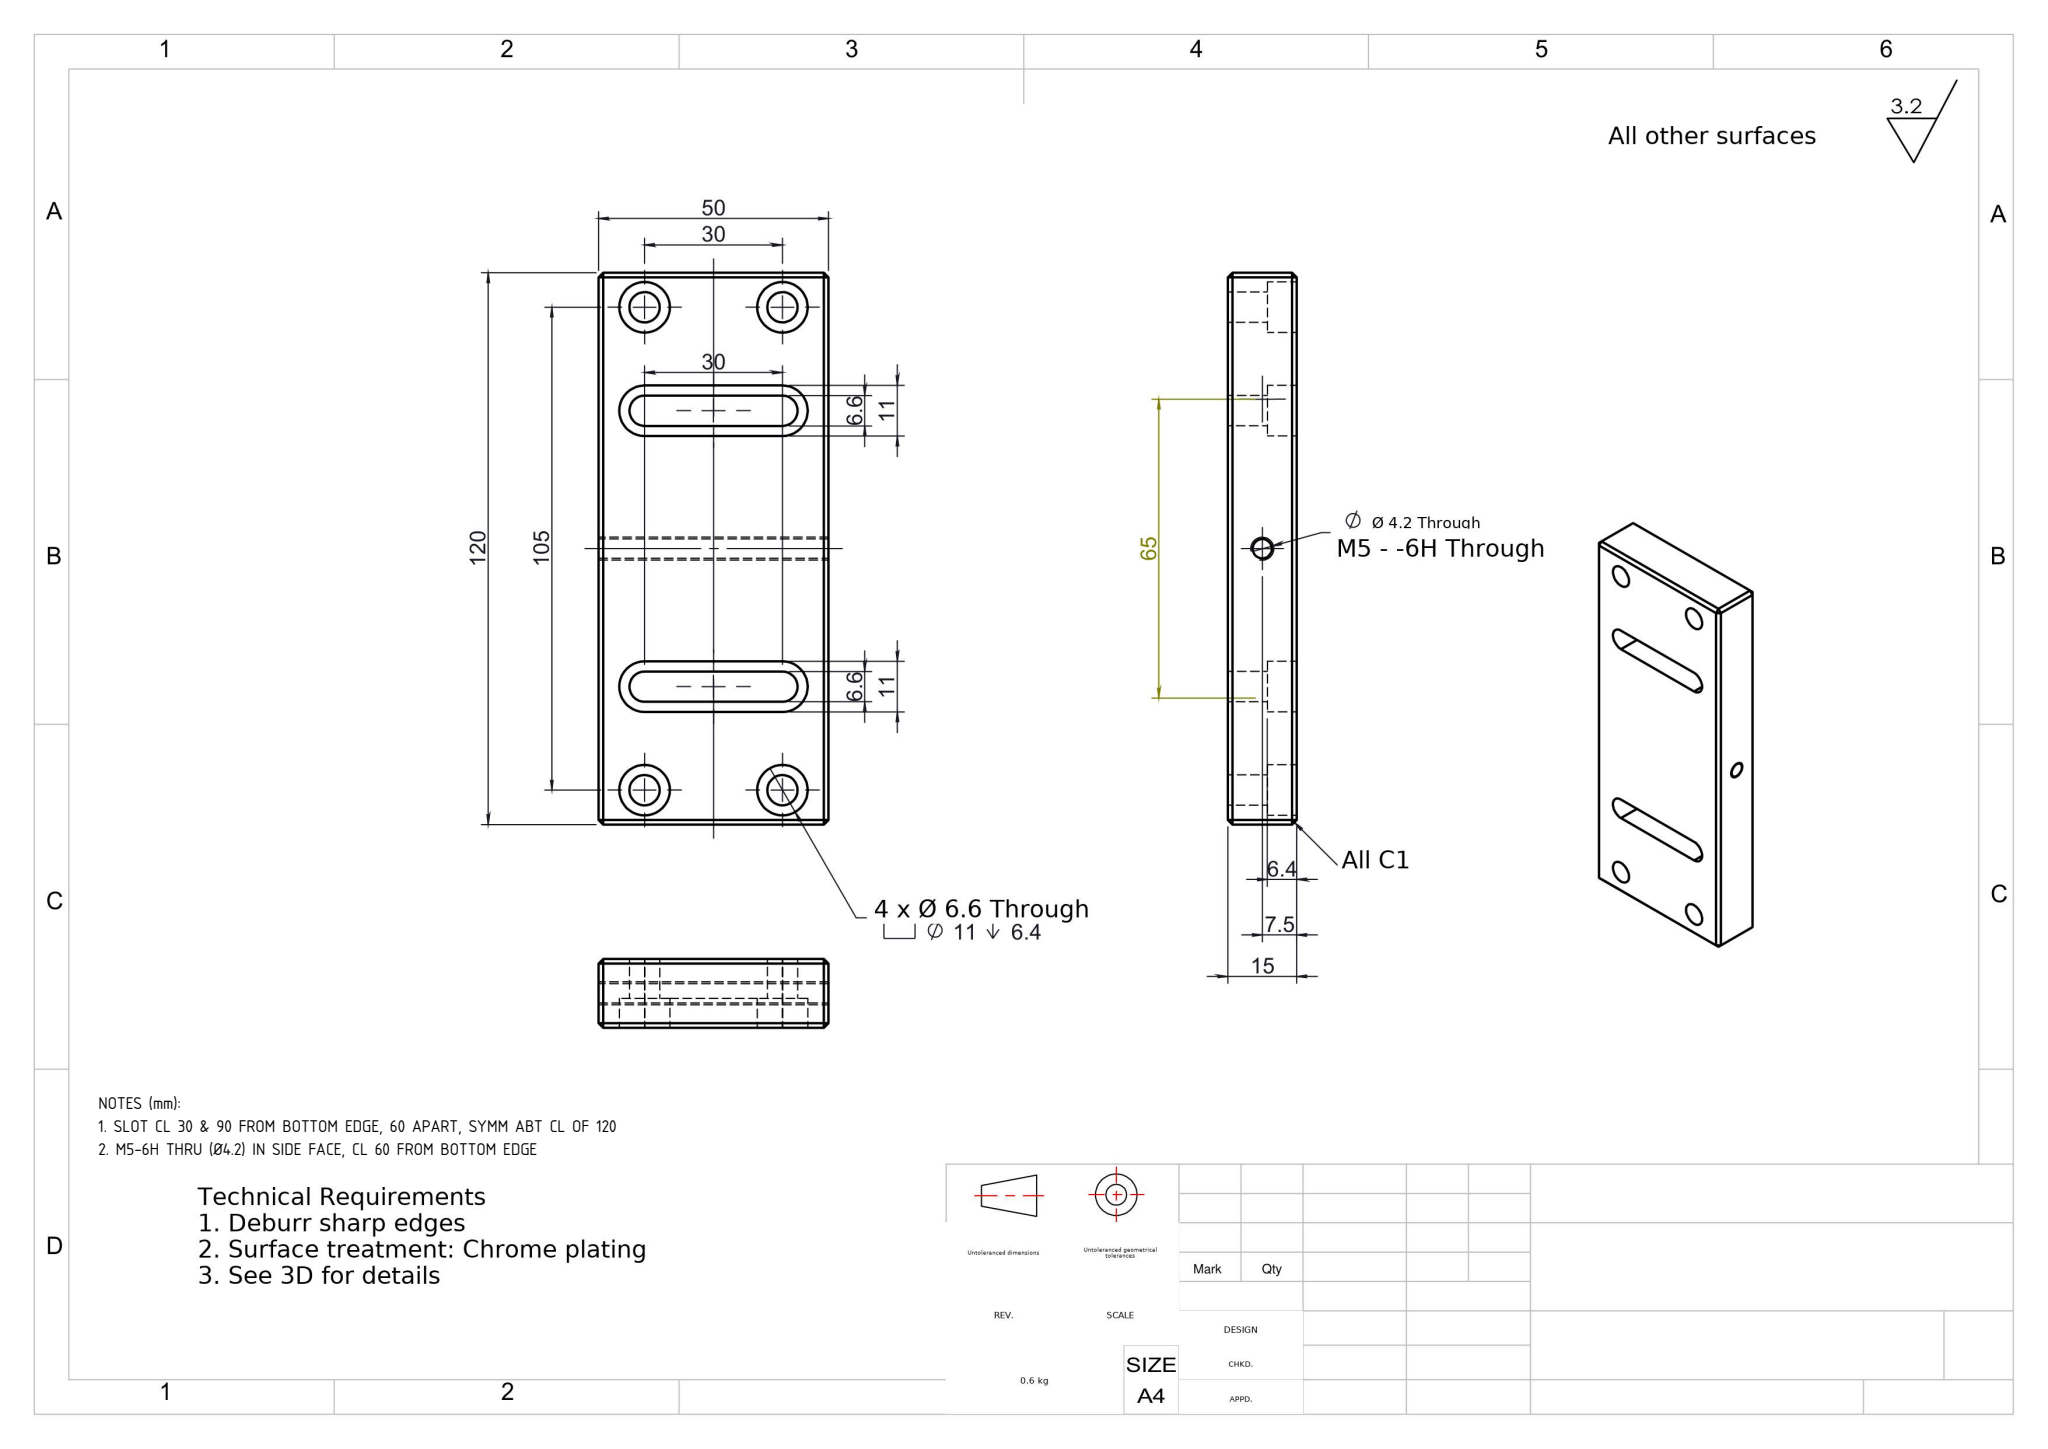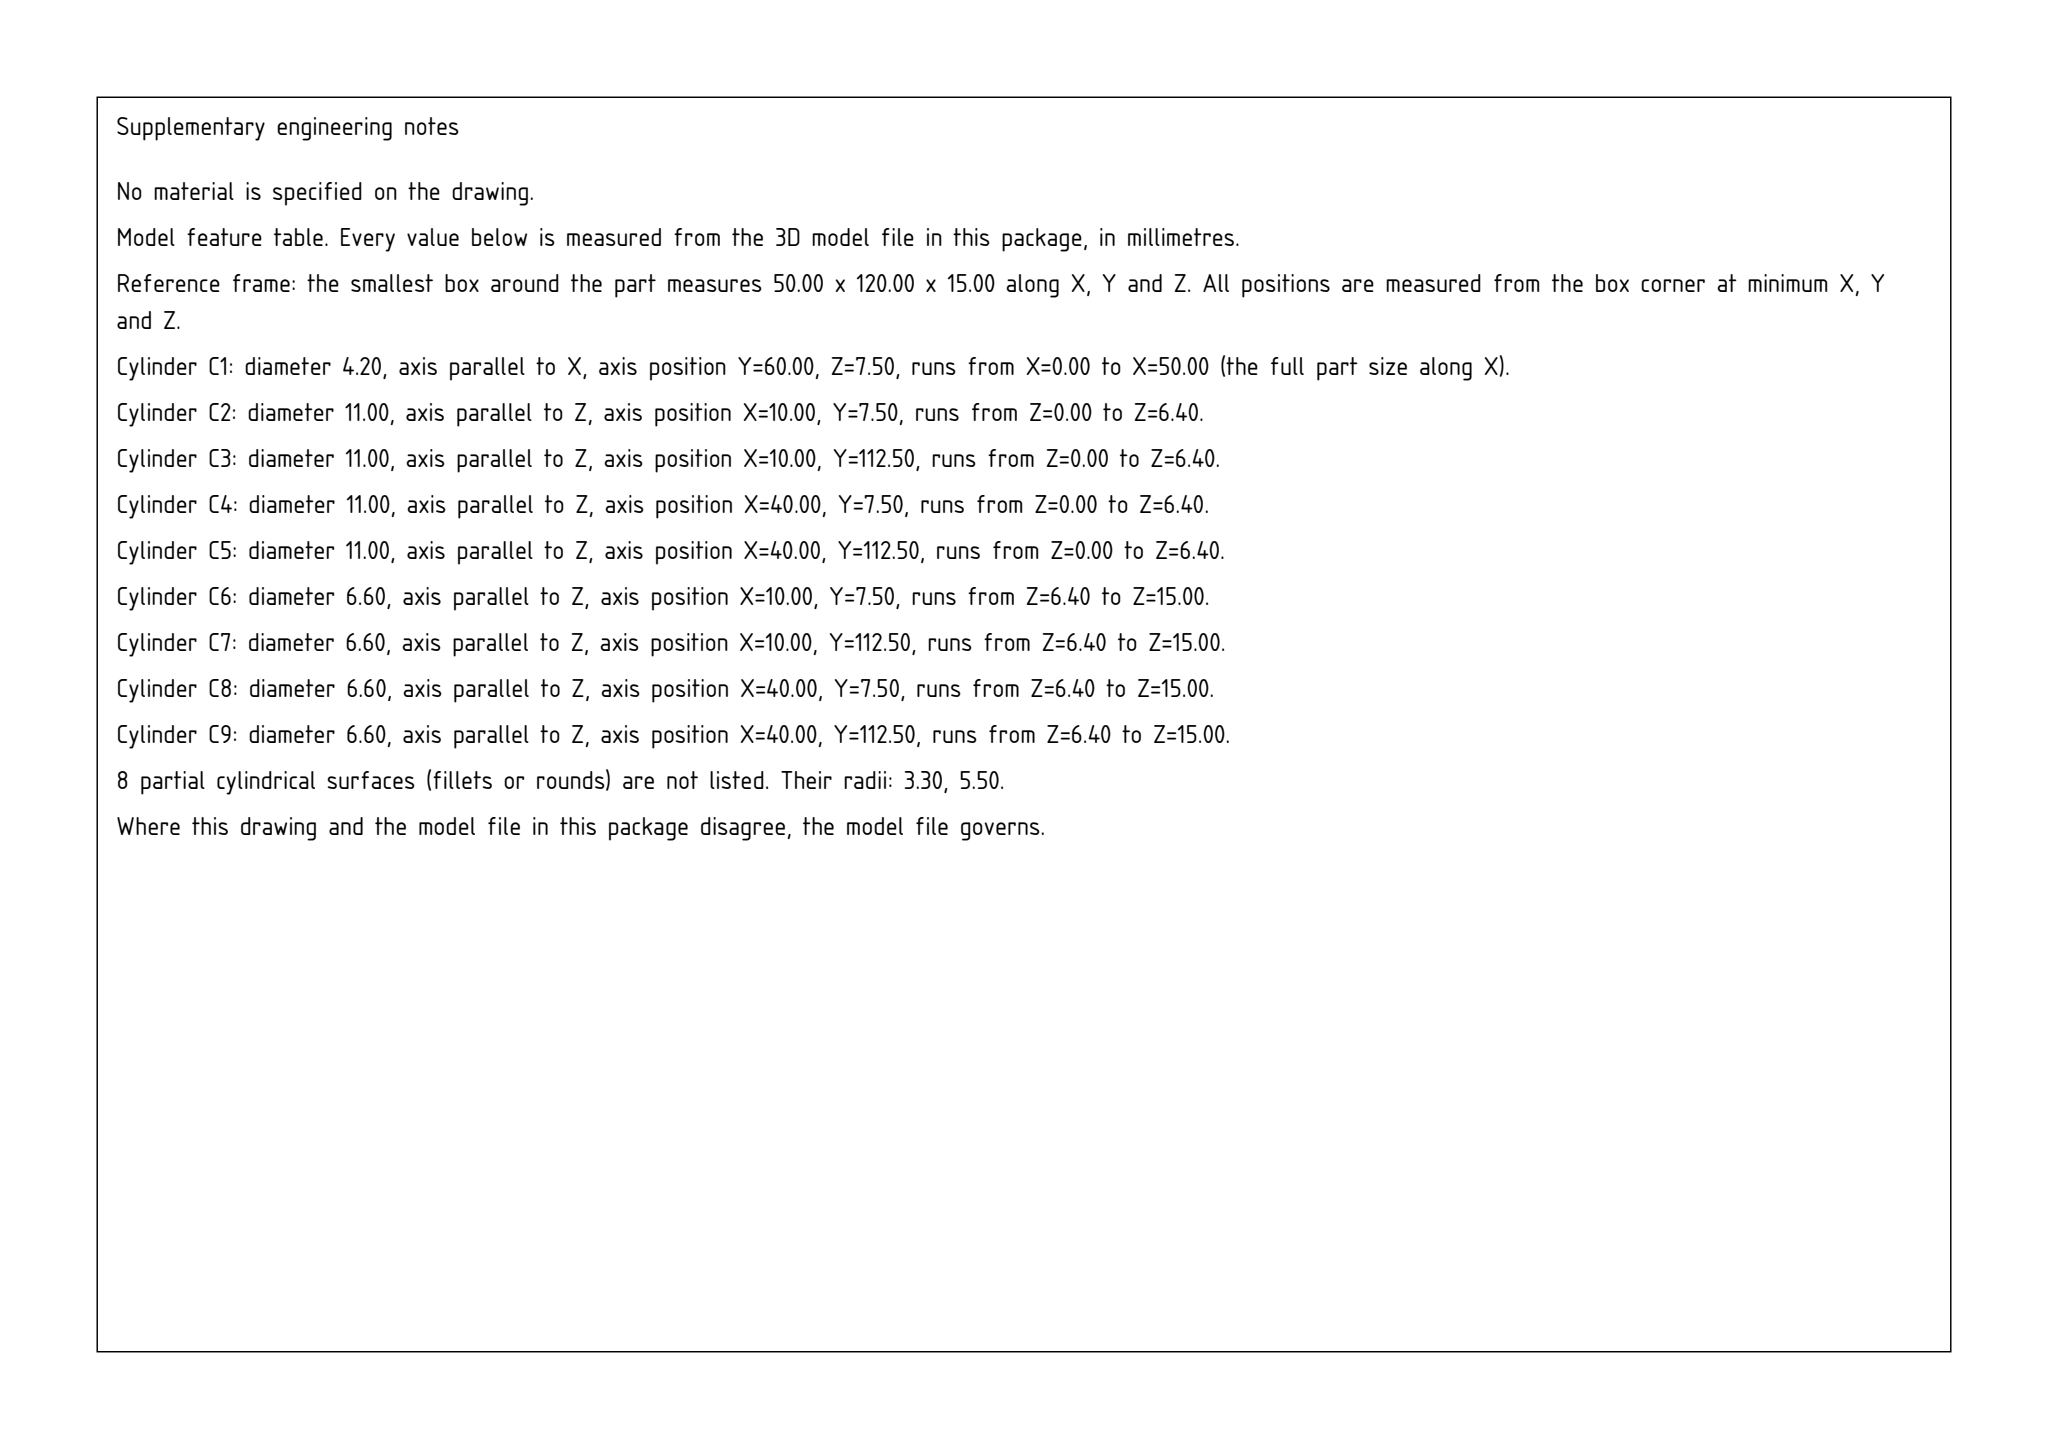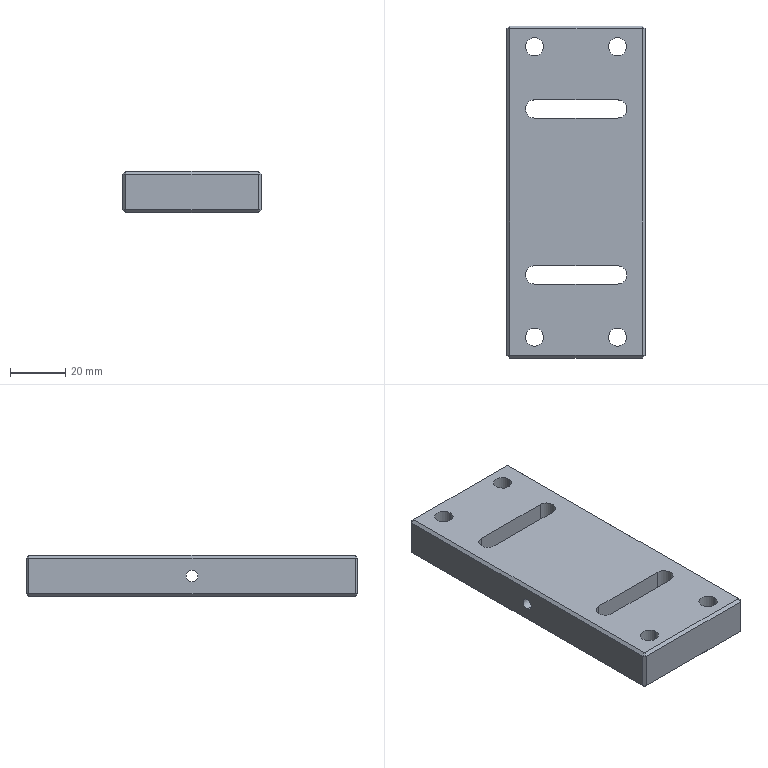Part | SolidWorks | mm | 1 solid | 70 faces | box 50 x 120 x 15 mm | volume 75898 mm3 | plane 40 | cylinder 30 | commonest cylinder face diameters 11 x14 6.6 x14 4.2 x2
Drawing notes:
SLOT CL 30 & 90 FROM BOTTOM EDGE, 60 APART, SYMM ABT CL OF 120 | from the solid: Slot end cyls Ø6.6/Ø11 at y=30 & y=90 (x=10 & 40); slot flats y=24.5-35.5 & 84.5-95.5
M5-6H THRU (Ø4.2) IN SIDE FACE, CL 60 FROM BOTTOM EDGE | from the solid: Ø4.2 cyl, axis x, pos y=60.0, z=7.5, length 50; bbox y=120 so y=60 is mid-height